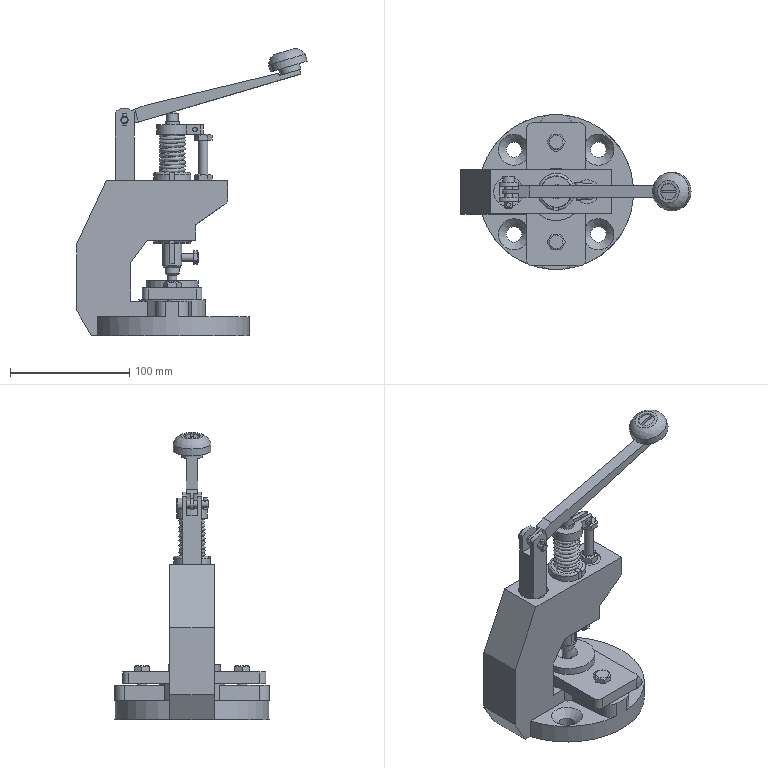Assembly | NX | mm | 21 component files | 21 solids | 306 faces | box 193.26 x 130 x 241.09 mm | volume 693469 mm3 | plane 180 | cylinder 82 | cone 33 | spline 7 | torus 2 | sphere 2 | commonest cylinder face diameters 8 x12 10 x9 4 x6 12 x5 13 x5 18 x5 7.785 x4 6 x4
Bill of materials:
unnamed part 1 | 1 |  | Long, slender rectangular bar with a short tab at each end that sticks out to one side, giving a shallow C or bracket profile.
unnamed part 2 | 1 |  | Several components merged into one model: a round flanged base with four countersunk holes and two plain holes; a raised plate with two lobes and a central round boss on top of the base; and an upright C-shaped block with an overhanging arm. The top of the arm has holes and a short cylindrical stub with a split or notched ring.
unnamed part 3 | 1 |  | Flat rectangular plate with rounded corners. It has a large central through-hole with a counterbore, a slotted hole near one end and a small round hole near the other end.
unnamed part 4 | 2 |  | Hex-head bolt-shaped part with a plain cylindrical shank and a chamfered tip.
unnamed part 5 | 1 |  | Hexagonal nut-shaped part with a central through-bore and chamfered corners on both faces.
unnamed part 6 | 1 |  | Solid cylindrical pin with steps along its length. It has a domed end, a narrow neck between two larger sections, and a slightly chamfered base.
unnamed part 7 | 1 |  | Solid round shaft with a larger collar part-way along. One side of the collar is flat and the other tapers down to the shaft.
unnamed part 8 | 1 |  | Screw-shaped part with a slotted round head (low, flat-topped) and a plain cylindrical shank with a chamfered end.
unnamed part 9 | 1 |  | Long thin-walled cylindrical tube with a small cross-hole through the wall near one end, plus small notches or features at the ends.
unnamed part 10 | 1 |  | Round knob-like part with a domed top, a cylindrical skirt and a smaller cylindrical boss underneath. A through-hole runs down the centre, with a counterbore or recess.
unnamed part 11 | 1 |  | Short hex-head bolt-shaped part with a plain cylindrical shank and a chamfered tip.
unnamed part 12 | 1 |  | Long hex-head bolt-shaped part with a slender plain cylindrical shank and a chamfered tip.
unnamed part 13 | 1 |  | Cylindrical helical coil of round-section wire with roughly constant diameter and pitch; the end coil is flattened into a flat annular face, similar to a compression spring.
unnamed part 14 | 1 |  | Headed cylindrical pin or screw-like part: a plain round shank with a chamfered tip and a larger cylindrical head with a slot cut into its end face.
unnamed part 15 | 1 |  | Plain solid cylinder (rod or pin blank) with flat ends.
unnamed part 16 | 1 |  | Rectangular fork (clevis-like) body: two parallel prongs with rounded tips and aligned cross holes, an open slot between the prongs, and a small stepped cylindrical stub at the other end.
unnamed part 17 | 1 |  | Long, slender, tapered flat bar or lever arm. One end has a rounded eye with a through hole; the other end steps down to a thinner pad with a hole and continues into a narrow tab.
unnamed part 18 | 1 |  | Headed cylindrical pin with chamfered head and tip edges and a single cross hole through the shank near the tip, similar in form to a clevis pin.
unnamed part 19 | 1 |  | Flat ring with a central bore and a radial slit that runs out through two parallel tabs. A cross hole passes through both tabs, and the tab ends are chamfered, similar to a split clamp collar.
unnamed part 20 | 1 |  | Stepped, flanged round bushing or washer: a larger-diameter flange on a smaller-diameter boss, with a central countersunk through hole.
Mates:
1. fix | base 1 component
2. concentric | base 1 edge | support 1 edge
3. parallel | support 1 face | base 1 face
4. touch align | SPRING_CYLINDER_COMPRESSION_1 1 datumaxis | base 1 face
5. touch align | base 1 face | SPRING_CYLINDER_COMPRESSION_1 1 face
6. touch align | retaining_ring 1 face | base 1 face
7. touch align | retaining_ring 1 face | SPRING_CYLINDER_COMPRESSION_1 1 face
8. parallel | retaining_ring 1 face | base 1 face
9. touch align | lever 1 face | support 1 face
10. center | lever 1 face | lever 1 face | support 1 face | support 1 face
11. touch align | ejector_pin 1 face | retaining_ring 1 face
12. touch align | lever 1 face | ejector_pin 1 face
13. concentric | screw_m4 1 | retaining_ring 1 edge
14. parallel | screw_m4 1 | base 1 face
15. concentric | lever 1 edge | handle 1 edge
16. concentric | screw_m8 1 edge | handle 1 edge
17. parallel | screw_m8 1 face | lever 1 face
18. concentric | base 1 edge | nut_m8 1 arc
19. parallel | nut_m8 1 | base 1 face
20. touch align | bolt_m8x45 1 face | nut_m8 1
21. touch align | bolt_m8x45 1 face | retaining_ring 1 face
22. parallel | bolt_m8x45 1 face | base 1 face
23. parallel | sleeve 1 face | base 1 face
24. touch align | bolt_m6x30 1 face | sleeve 1 face
25. concentric | punch 1 edge | sleeve 1 edge
26. center | key 1 face | key 1 face | base 1 face | base 1 face
27. touch align | key 1 face | base 1 face
28. touch align | clamp_plate 1 face | base 1 face
29. touch align | clamp_plate 1 face | base 1 face
30. parallel | clamp_plate 1 face | base 1 face
31. concentric | punching_die 1 edge | clamp_plate 1 arc
32. concentric | clamp_plate 1 edge | bolt_m8x35 2 edge
33. parallel | bolt_m8x35 2 face | clamp_plate 1 face
34. parallel | bolt_m8x35 1 face | bolt_m8x35 2 face
35. concentric | dowel_pin 1 arc | support 1 edge
36. touch align | pin 1 | dowel_pin 1
37. distance | pin 1 | dowel_pin 1
38. concentric | sleeve 1 edge | ejector_pin 1 edge